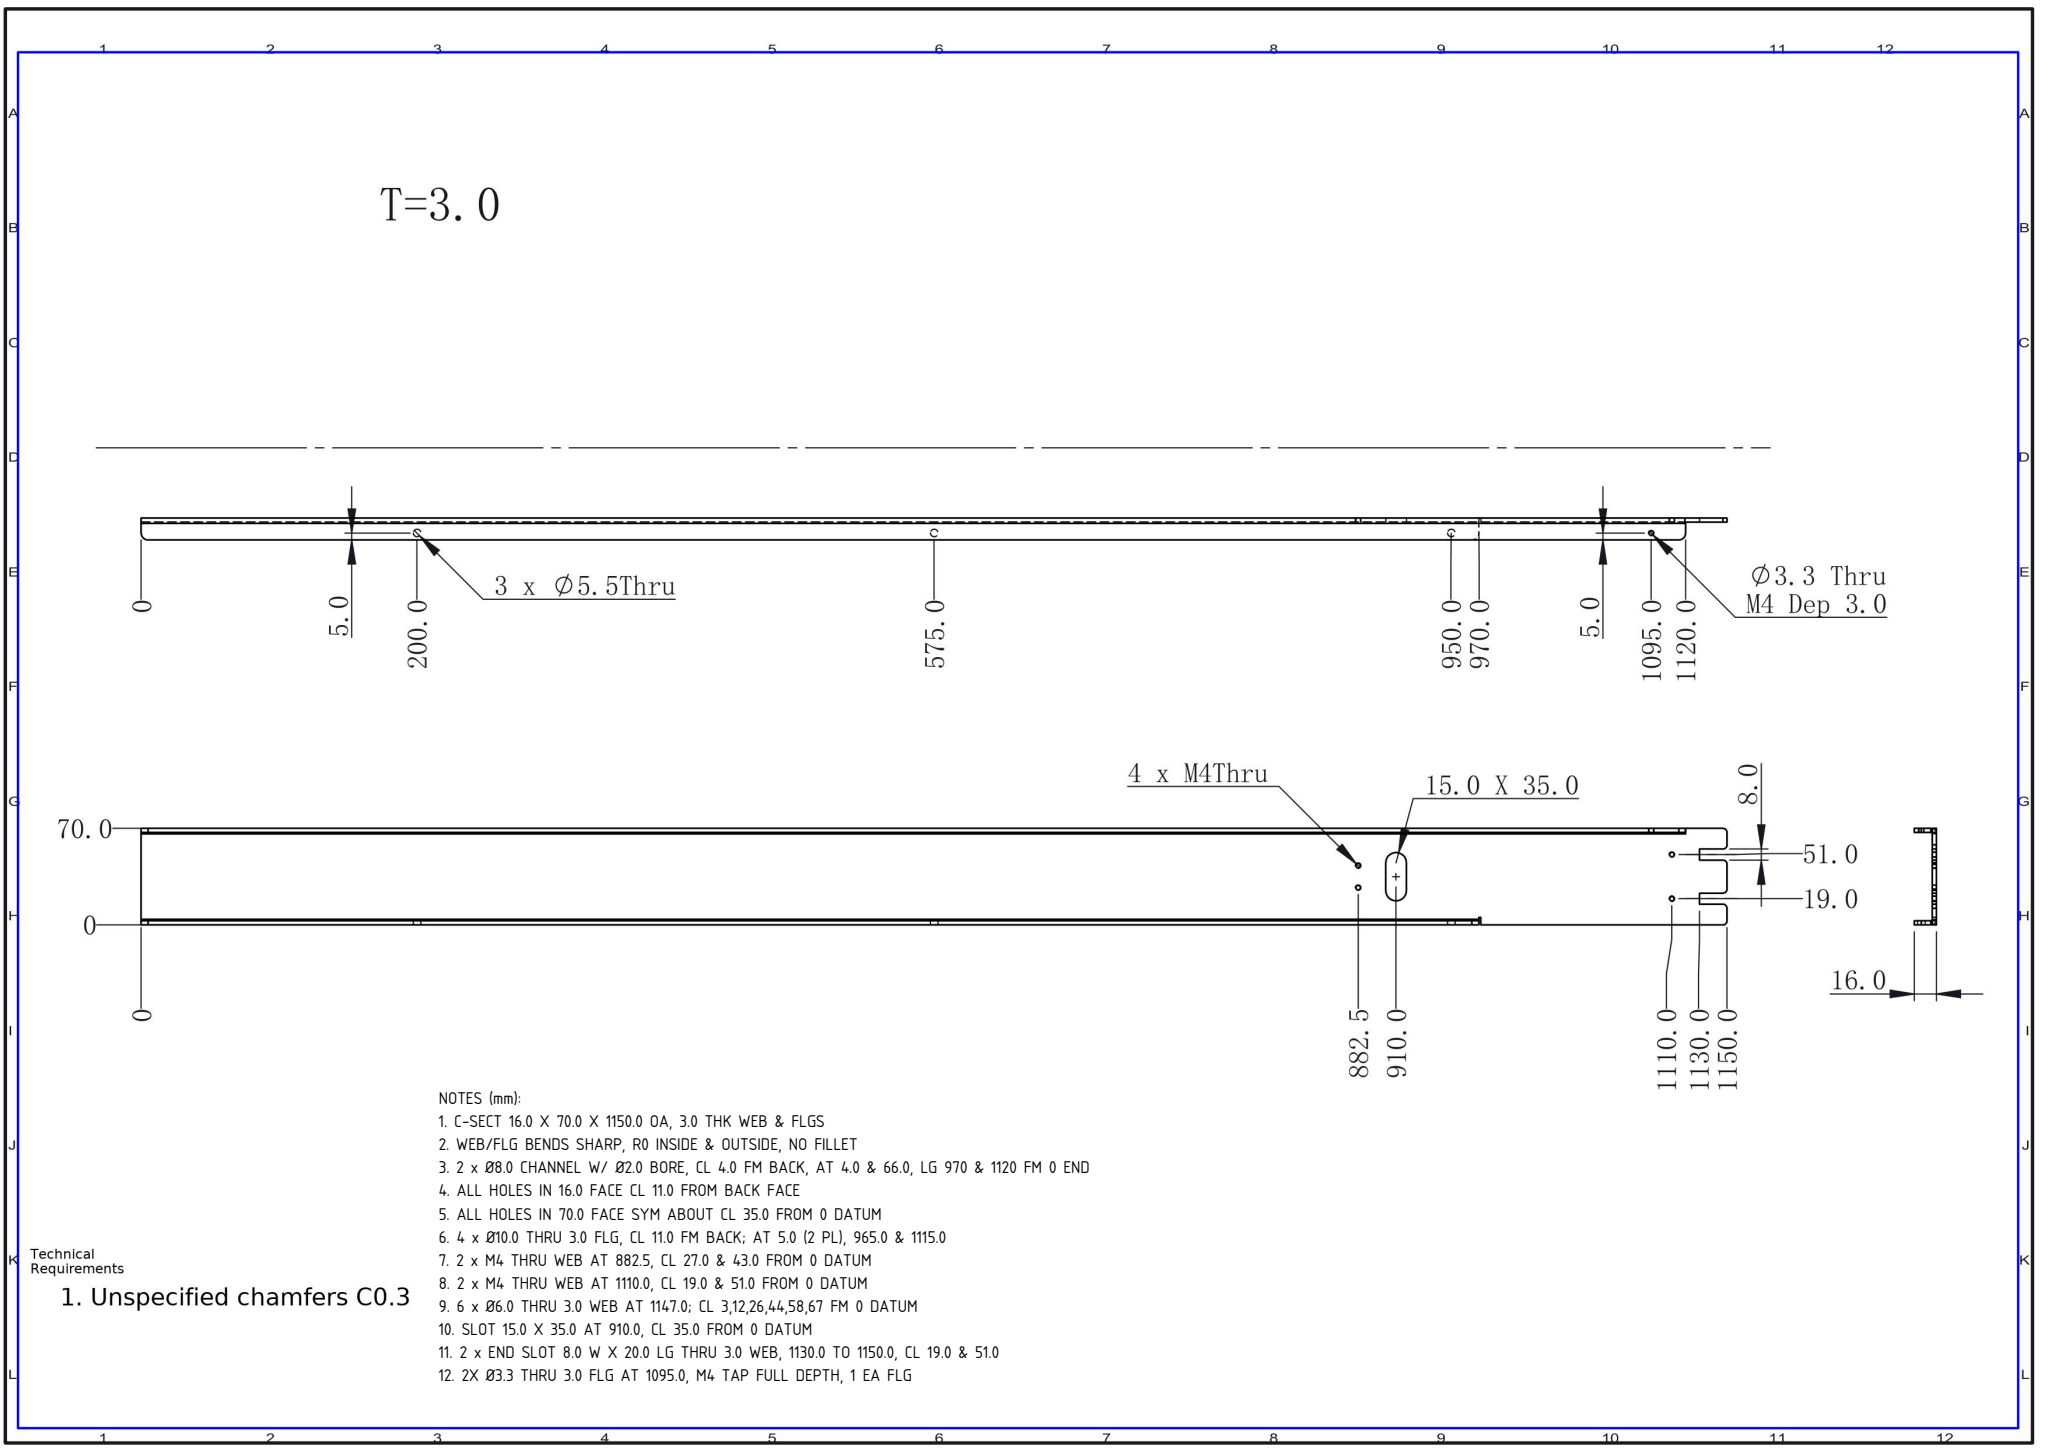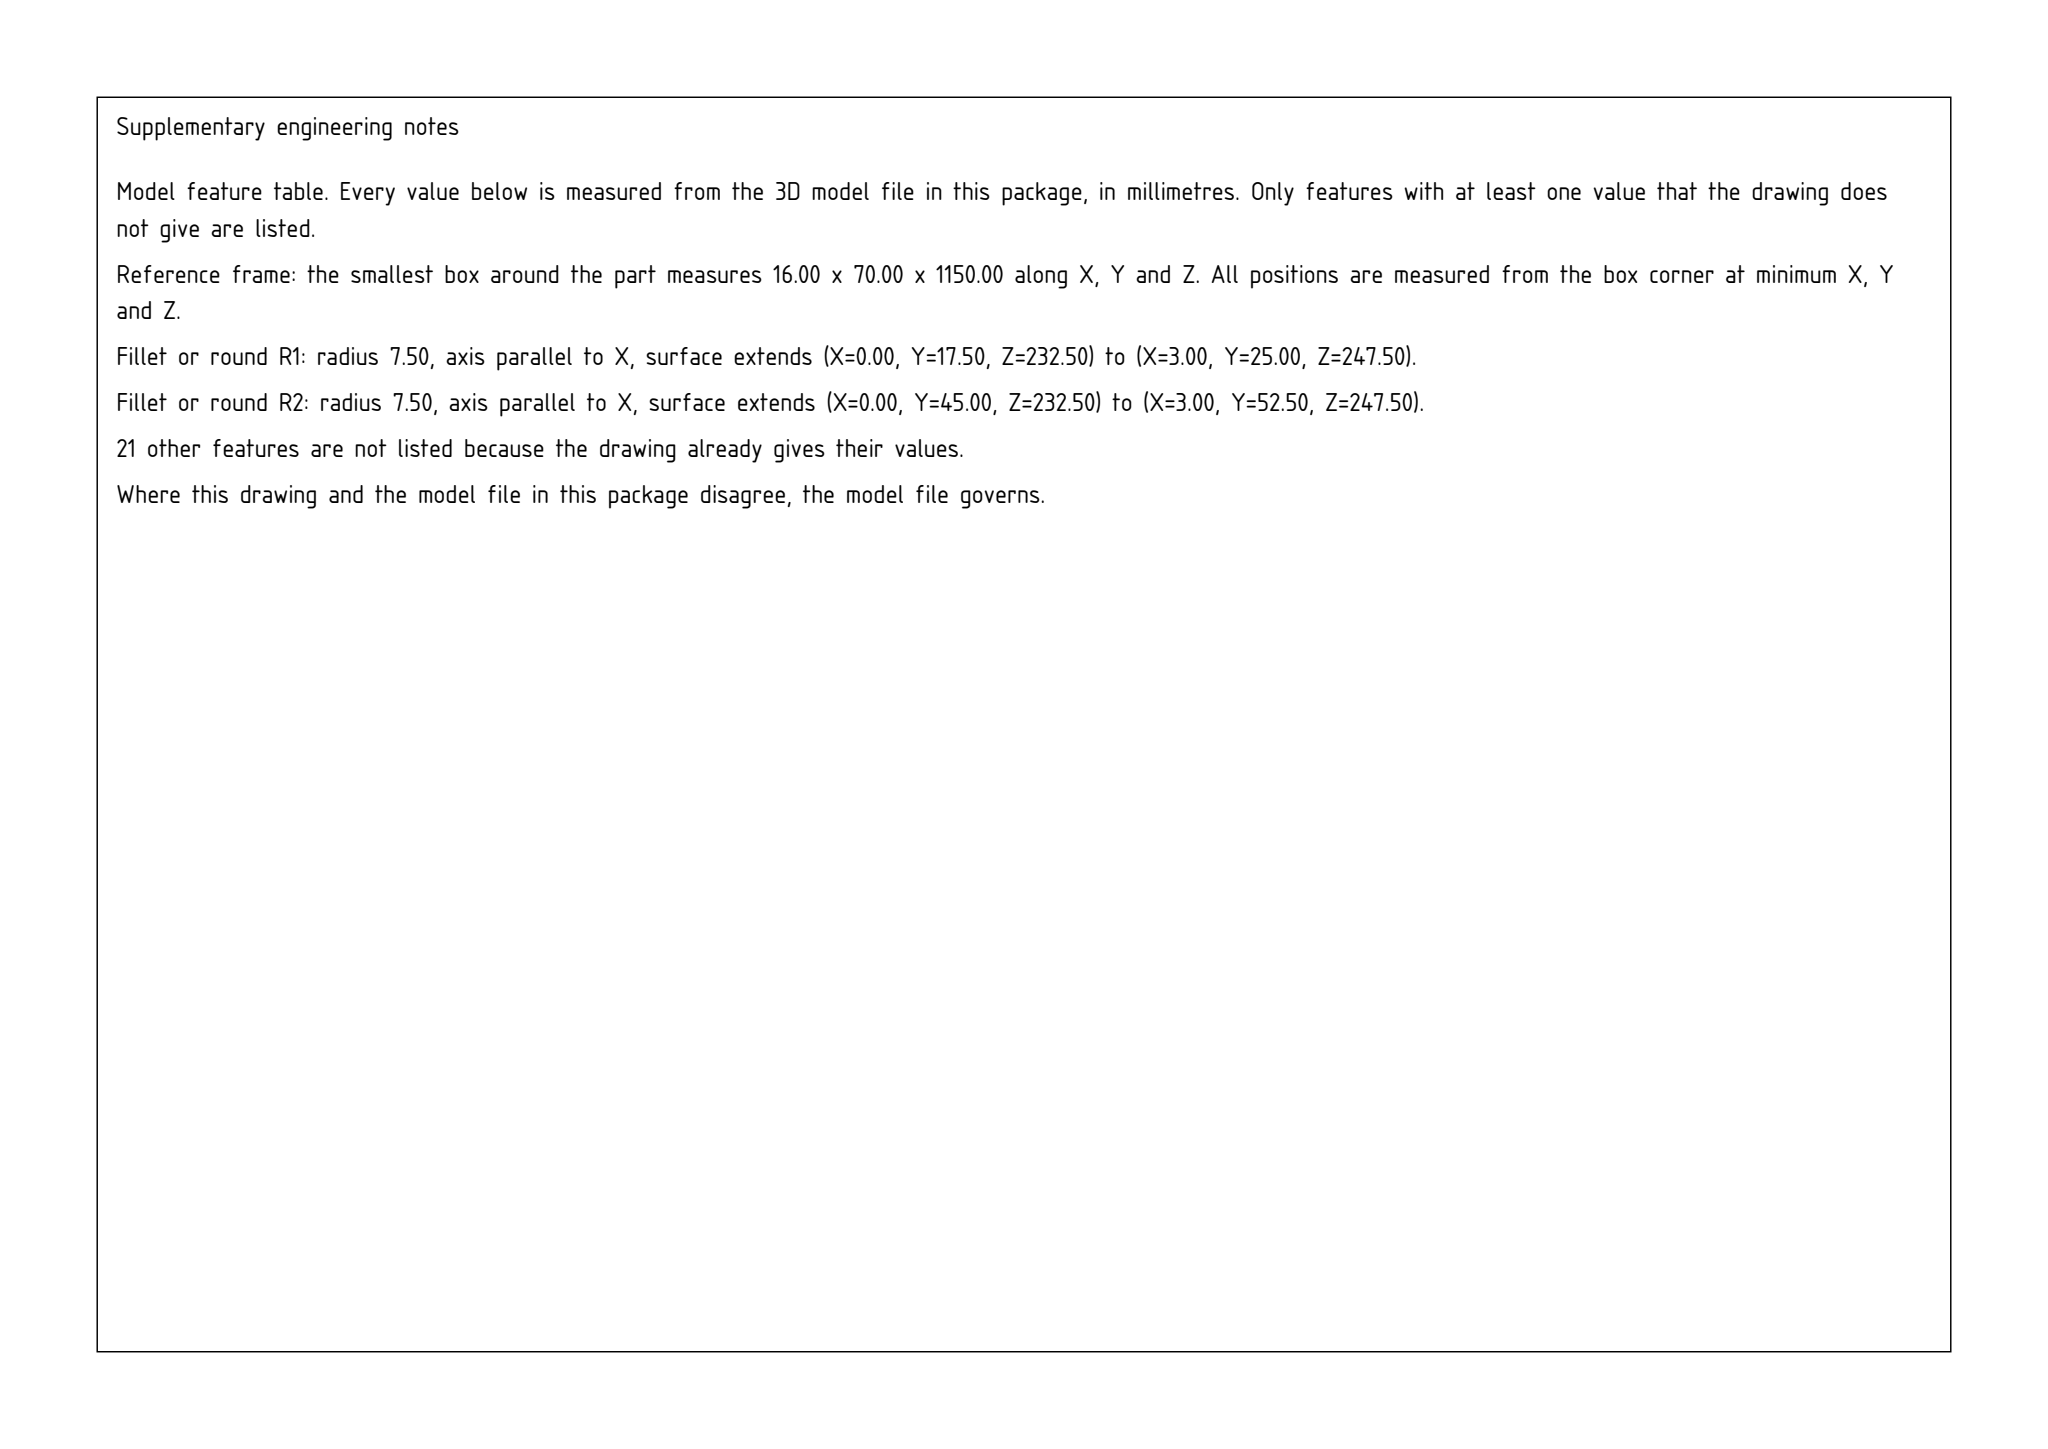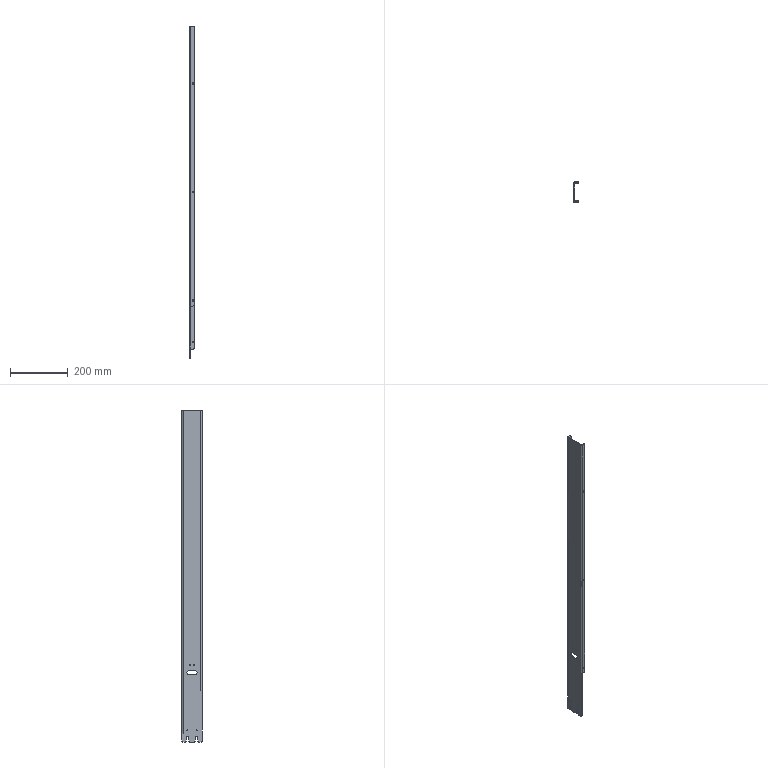Part | SolidWorks | mm | 1 solid | 66 faces | box 16 x 70 x 1150 mm | volume 313428 mm3 | plane 34 | cylinder 32 | commonest cylinder face diameters 3.3 x10 5.5 x6 6 x6 10 x4 8 x2 2 x2 15 x2
Drawing notes:
C-SECT 16.0 X 70.0 X 1150.0 OA, 3.0 THK WEB & FLGS | from the solid: bbox 16x70x1150; x planes 0,3,16; y planes 0,3,67,70
WEB/FLG BENDS SHARP, R0 INSIDE & OUTSIDE, NO FILLET | from the solid: fillet_radii empty; planes x=0,3,16 / y=0,3,67,70 meet square
2 x Ø8.0 CHANNEL W/ Ø2.0 BORE, CL 4.0 FM BACK, AT 4.0 & 66.0, LG 970 & 1120 FM 0 END | from the solid: Ø8.0 & Ø2.0 z-axis cyls at (4,4) L970 and (4,66) L1120, start z=0
ALL HOLES IN 16.0 FACE CL 11.0 FROM BACK FACE | from the solid: all y-axis cyls Ø5.5, Ø3.3, Ø10 at x=11.0 of 16.0 width
ALL HOLES IN 70.0 FACE SYM ABOUT CL 35.0 FROM 0 DATUM | from the solid: x-axis holes at y=19/51, 25/45, 27/43, 3/67, 12/58, 26/44
4 x Ø10.0 THRU 3.0 FLG, CL 11.0 FM BACK; AT 5.0 (2 PL), 965.0 & 1115.0 | from the solid: Ø10 y-axis cyls L3.0 at x=11.0, z=1145 (x2), 185, 35
2 x M4 THRU WEB AT 882.5, CL 27.0 & 43.0 FROM 0 DATUM | from the solid: Ø3.3 x-axis cyls at y=27 & 43, z=267.5 (=1150-882.5), L=3.0
2 x M4 THRU WEB AT 1110.0, CL 19.0 & 51.0 FROM 0 DATUM | from the solid: Ø3.3 x-axis cyls at y=19 & 51, z=40 (=1150-1110), L=3.0
6 x Ø6.0 THRU 3.0 WEB AT 1147.0; CL 3,12,26,44,58,67 FM 0 DATUM | from the solid: Ø6.0 x-axis cyls L3.0 at z=3.0 (=1147.0), y=3,12,26,44,58,67
SLOT 15.0 X 35.0 AT 910.0, CL 35.0 FROM 0 DATUM | from the solid: Ø15 x-axis cyls at y=25 & 45, z=240 (=910); slot 35 in Y, 15 in Z
2 x END SLOT 8.0 W X 20.0 LG THRU 3.0 WEB, 1130.0 TO 1150.0, CL 19.0 & 51.0 | from the solid: y planes 15/23 & 47/55 (8.0 W), z planes 20 & 0 (=1130 & 1150), x 0-3
2X Ø3.3 THRU 3.0 FLG AT 1095.0, M4 TAP FULL DEPTH, 1 EA FLG | from the solid: cylinders 3.3 dia, axis y, [x=11, z=55], length 3.0, count 2 -> 1150-55 = 1095.0 from left datum; length 3.0 = flange thickness, so tap is full depth of one 3.0 flange, not 'Thru + Dep 3.0'